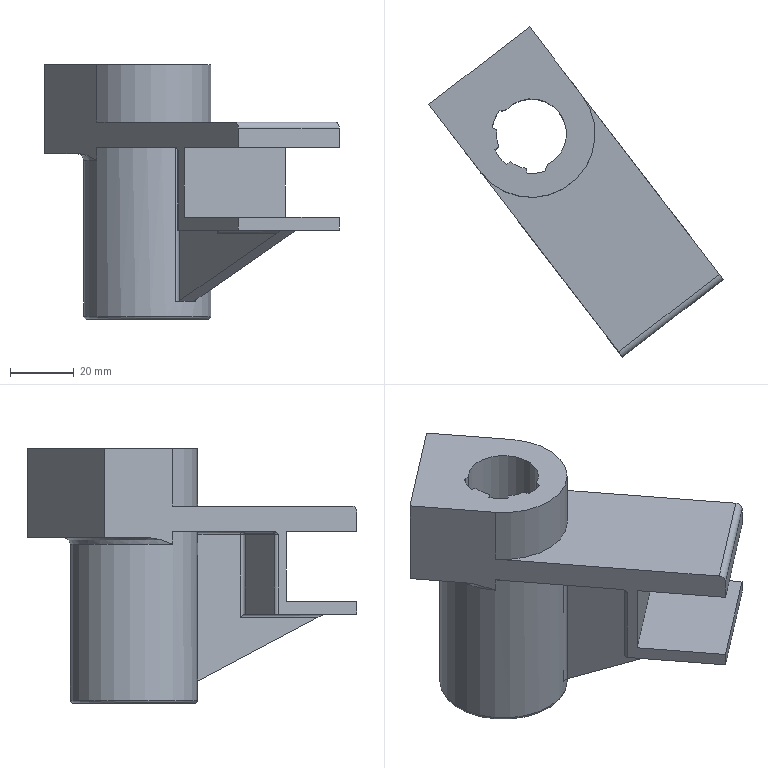Component | NX | CA6140-ZHOU12-BOCHA2 | 1 solid | 58 faces | volume 114380 mm3 | plane 29 | cylinder 21 | torus 5 | sphere 3 | commonest cylinder face diameters 2 x12 22 x3 25 x3 40 x2 4 x1